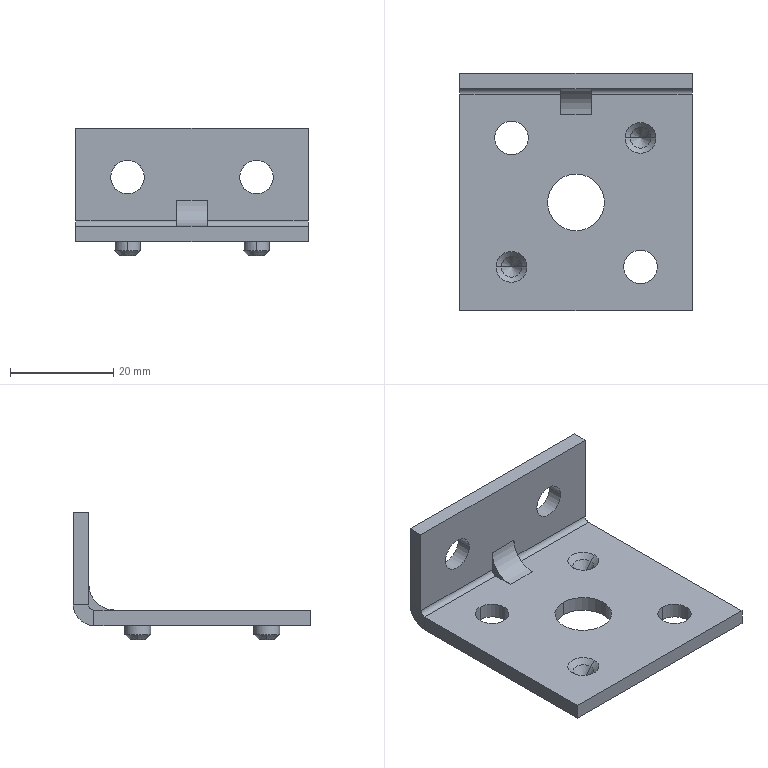Component | SolidWorks | Bracket(No.11)-1 | 1 solid | 52 faces | volume 7955 mm3 | plane 21 | cylinder 19 | cone 12 | commonest cylinder face diameters 6.5 x8 5 x4 11 x2 8 x2 2 x2 10 x1